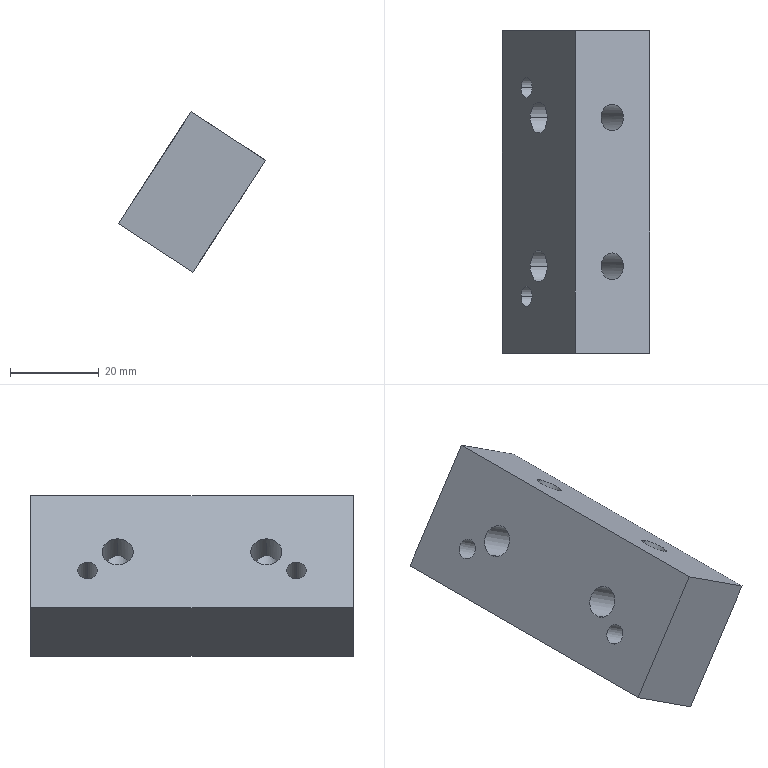Component | SolidWorks | DischargePortPushRodFixingPlate-1 | 1 solid | 34 faces | box 33.11 x 72.6 x 36.05 mm | volume 40398 mm3 | cylinder 22 | plane 12 | commonest cylinder face diameters 6 x10 8 x4 4.5 x4 7 x4
build123d program:
from build123d import *

# Parameters (mm, degrees)
SKETCH1_W                                         = 72.6
SKETCH1_H                                         = 30
BOSS_EXTRUDE1_DEPTH                               = 20
F_7_0_7_DIAMETER_HOLE1_D                          = 7
HOLE_SIZE_ACCORDING_TO_TYPE_OF_HEX_SO_D           = 4.5
HOLE_SIZE_ACCORDING_TO_TYPE_OF_HEX_SO_CBORE_D     = 8
HOLE_SIZE_ACCORDING_TO_TYPE_OF_HEX_SO_CBORE_DEPTH = 4.6
M6_TAPPED_HOLE1_D                                 = 6
M6_TAPPED_HOLE1_DEPTH                             = 17


with BuildPart() as part:
    # Sketch1 → Boss-Extrude1 (new body)
    with BuildSketch(Plane(origin=(0, 0, 0), x_dir=(1, 0, 0), z_dir=(0, 1, 0))):
        Rectangle(SKETCH1_W, SKETCH1_H)
    extrude(amount=BOSS_EXTRUDE1_DEPTH)

    # 7.0 _7_ Diameter Hole1 (through all)
    with Locations(Plane(origin=(-16.75, 0, 0), x_dir=(0, 0, -1), z_dir=(0, -1, 0))):
        with Locations((0, 0)):
            f_7_0_7_diameter_hole1 = Hole(F_7_0_7_DIAMETER_HOLE1_D / 2)

    # Mirror1: 7.0 _7_ Diameter Hole1 across plane
    add(f_7_0_7_diameter_hole1.mirror(Plane(origin=(0, 0, 0), x_dir=(0, 0, 1), z_dir=(1, 0, 0))), mode=Mode.SUBTRACT)

    # Hole Size _ according to_ type of Hex So (through all)
    with Locations(Plane(origin=(23.5, 20, -5.001), x_dir=(0, 0, 1), z_dir=(0, 1, 0))):
        with Locations((0, 0), (0.0006475, -47)):
            CounterBoreHole(HOLE_SIZE_ACCORDING_TO_TYPE_OF_HEX_SO_D / 2, HOLE_SIZE_ACCORDING_TO_TYPE_OF_HEX_SO_CBORE_D / 2, HOLE_SIZE_ACCORDING_TO_TYPE_OF_HEX_SO_CBORE_DEPTH)

    # M6 Tapped Hole1
    with Locations(Plane(origin=(16.75, 10, 15), x_dir=(1, 0, 0), z_dir=(0, 0, 1))):
        with Locations((0, 0)):
            m6_tapped_hole1 = Hole(M6_TAPPED_HOLE1_D / 2, depth=M6_TAPPED_HOLE1_DEPTH)

    # Mirror2: M6 Tapped Hole1 across plane
    add(m6_tapped_hole1.mirror(Plane(origin=(0, 0, 0), x_dir=(0, 0, 1), z_dir=(1, 0, 0))), mode=Mode.SUBTRACT)


solid = part.part

# Placed as in the assembly
solid = solid.moved(Location((100.9, -0.384, 277.991), (0, 33, -90)))